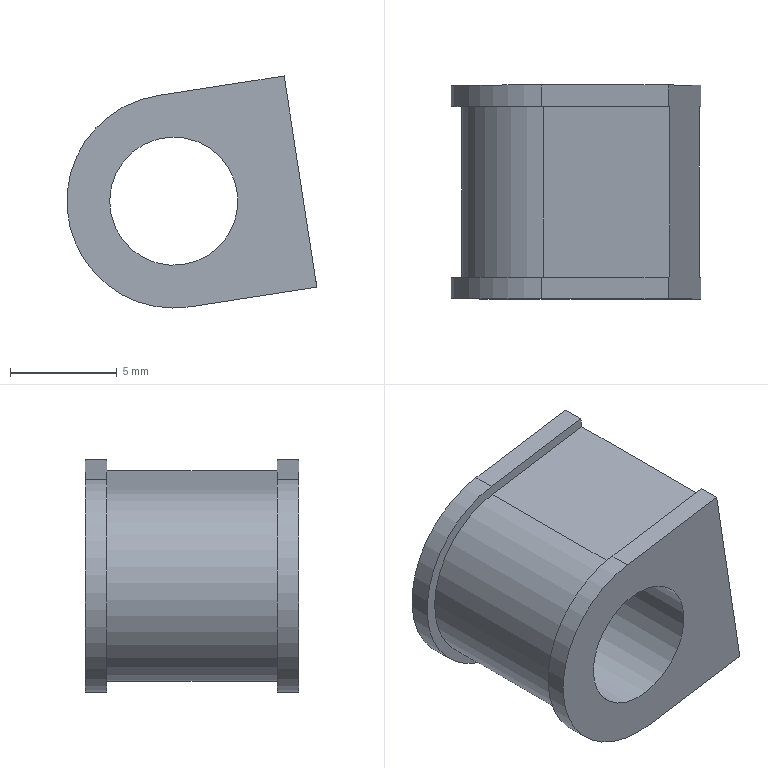Component | NX | SMALL_CONN_BLOCK | 1 solid | 15 faces | volume 602 mm3 | plane 11 | cylinder 4 | commonest cylinder face diameters 10 x2 9 x1 6 x1